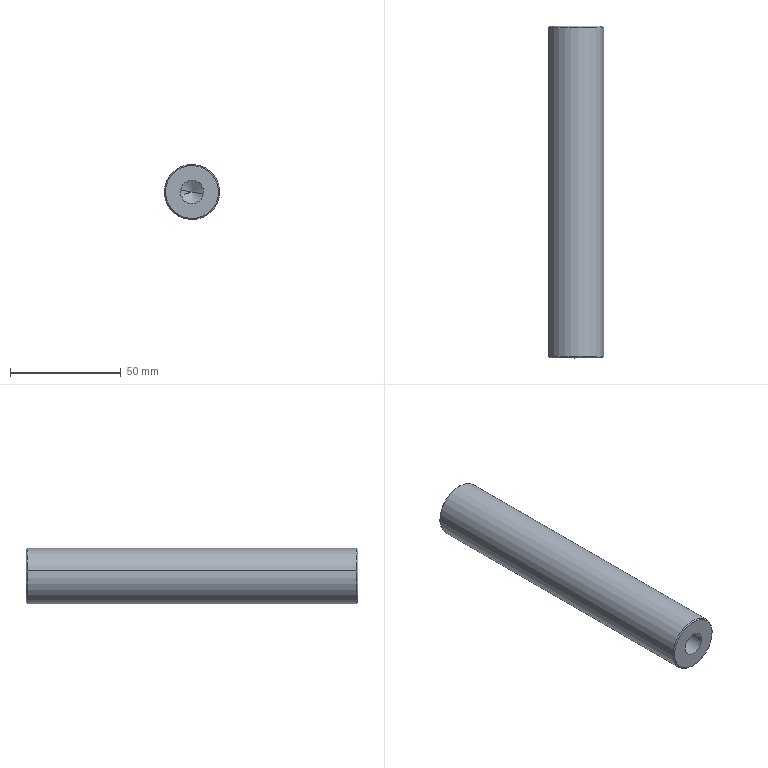Component | SolidWorks | 002AS-20130718-1_011A-20130717-4 | 1 solid | 16 faces | box 25 x 150 x 25 mm | volume 68494 mm3 | cone 8 | cylinder 6 | plane 2 | commonest cylinder face diameters 10.5 x4 25 x2
build123d program:
from build123d import *

# Parameters (mm, degrees)
SKETCH1_R                  = 12.5
BOSS_EXTRUDE1_DEPTH        = 150
M12X1_5_TAPPED_HOLE1_D     = 10.5
M12X1_5_TAPPED_HOLE1_DEPTH = 28.5
M12X1_5_TAPPED_HOLE1_TIP   = 3.155
M12X1_5_TAPPED_HOLE2_D     = 10.5
M12X1_5_TAPPED_HOLE2_DEPTH = 28.5
M12X1_5_TAPPED_HOLE2_TIP   = 3.155
CHAMFER1_SIZE              = 0.5


with BuildPart() as part:
    # Sketch1 → Boss-Extrude1 (new body)
    with BuildSketch(Plane(origin=(0, 0, 0), x_dir=(1, 0, 0), z_dir=(0, 1, 0))):
        with Locations(Location((0, 0, 0), (0, 0, 270))):
            Circle(SKETCH1_R)
    extrude(amount=BOSS_EXTRUDE1_DEPTH)

    # M12x1.5 Tapped Hole1
    with Locations(Plane.ZX.offset(150)):
        with Locations((0, 0)):
            Hole(M12X1_5_TAPPED_HOLE1_D / 2, depth=M12X1_5_TAPPED_HOLE1_DEPTH)
            with Locations((0, 0, -(M12X1_5_TAPPED_HOLE1_DEPTH + M12X1_5_TAPPED_HOLE1_TIP / 2))):  # 118° drill point
                Cone(0, M12X1_5_TAPPED_HOLE1_D / 2, M12X1_5_TAPPED_HOLE1_TIP, mode=Mode.SUBTRACT)

    # M12x1.5 Tapped Hole2
    with Locations(Plane(origin=(0, 0, 0), x_dir=(0, 0, -1), z_dir=(0, -1, 0))):
        with Locations((0, 0)):
            Hole(M12X1_5_TAPPED_HOLE2_D / 2, depth=M12X1_5_TAPPED_HOLE2_DEPTH)
            with Locations((0, 0, -(M12X1_5_TAPPED_HOLE2_DEPTH + M12X1_5_TAPPED_HOLE2_TIP / 2))):  # 118° drill point
                Cone(0, M12X1_5_TAPPED_HOLE2_D / 2, M12X1_5_TAPPED_HOLE2_TIP, mode=Mode.SUBTRACT)

    # Chamfer1
    chamfer1_edges = [part.edges().sort_by_distance(p)[0] for p in [
        (0, 0, -12.5),
        (0, 150, -12.5),
    ]]
    chamfer(chamfer1_edges, length=CHAMFER1_SIZE)


solid = part.part

# Placed as in the assembly
solid = solid.moved(Location((-292.1, 427.678, 29.291), (0, 0, 0)))
STEP:
#1=CARTESIAN_POINT('',(-11.036,16.838,1.066));
#2=VERTEX_POINT('',#1);
#3=CARTESIAN_POINT('',(-11.964,16.838,1.24));
#4=VERTEX_POINT('',#3);
#5=CARTESIAN_POINT('',(-11.5,16.838,1.153));
#6=DIRECTION('',(-0.,-1.,0.));
#7=DIRECTION('',(-0.9828,0.,0.1846));
#8=AXIS2_PLACEMENT_3D('',#5,#6,#7);
#9=CIRCLE('',#8,0.4724);
#10=EDGE_CURVE('',#2,#4,#9,.T.);
#11=ORIENTED_EDGE('',*,*,#10,.F.);
#12=CARTESIAN_POINT('',(-11.016,16.857,1.062));
#13=VERTEX_POINT('',#12);
#14=CARTESIAN_POINT('',(-11.016,16.857,1.062));
#15=DIRECTION('',(0.695,0.7071,-0.1305));
#16=VECTOR('',#15,39.37);
#17=LINE('',#14,#16);
#18=EDGE_CURVE('',#2,#13,#17,.T.);
#19=ORIENTED_EDGE('',*,*,#18,.T.);
#20=CARTESIAN_POINT('',(-11.984,16.857,1.244));
#21=VERTEX_POINT('',#20);
#22=CARTESIAN_POINT('',(-11.5,16.857,1.153));
#23=DIRECTION('',(0.,1.,-0.));
#24=DIRECTION('',(-0.9828,0.,0.1846));
#25=AXIS2_PLACEMENT_3D('',#22,#23,#24);
#26=CIRCLE('',#25,0.4921);
#27=EDGE_CURVE('',#21,#13,#26,.T.);
#28=ORIENTED_EDGE('',*,*,#27,.F.);
#29=CARTESIAN_POINT('',(-11.984,16.857,1.244));
#30=DIRECTION('',(-0.695,0.7071,0.1305));
#31=VECTOR('',#30,39.37);
#32=LINE('',#29,#31);
#33=EDGE_CURVE('',#4,#21,#32,.T.);
#34=ORIENTED_EDGE('',*,*,#33,.F.);
#35=EDGE_LOOP('',(#11,#19,#28,#34));
#36=FACE_OUTER_BOUND('',#35,.T.);
#37=CARTESIAN_POINT('',(-11.5,16.857,1.153));
#38=DIRECTION('',(0.,1.,-0.));
#39=DIRECTION('',(-0.9828,0.,0.1846));
#40=AXIS2_PLACEMENT_3D('',#37,#38,#39);
#41=CONICAL_SURFACE('',#40,0.4921,0.7854);
#42=ADVANCED_FACE('',(#36),#41,.T.);
#43=CARTESIAN_POINT('',(-11.964,22.743,1.24));
#44=VERTEX_POINT('',#43);
#45=CARTESIAN_POINT('',(-11.036,22.743,1.066));
#46=VERTEX_POINT('',#45);
#47=CARTESIAN_POINT('',(-11.5,22.743,1.153));
#48=DIRECTION('',(0.,1.,-0.));
#49=DIRECTION('',(-0.9828,0.,0.1846));
#50=AXIS2_PLACEMENT_3D('',#47,#48,#49);
#51=CIRCLE('',#50,0.4724);
#52=EDGE_CURVE('',#44,#46,#51,.T.);
#53=ORIENTED_EDGE('',*,*,#52,.F.);
#54=CARTESIAN_POINT('',(-11.984,22.724,1.244));
#55=VERTEX_POINT('',#54);
#56=CARTESIAN_POINT('',(-11.964,22.743,1.24));
#57=DIRECTION('',(-0.695,-0.7071,0.1305));
#58=VECTOR('',#57,39.37);
#59=LINE('',#56,#58);
#60=EDGE_CURVE('',#44,#55,#59,.T.);
#61=ORIENTED_EDGE('',*,*,#60,.T.);
#62=CARTESIAN_POINT('',(-11.016,22.724,1.062));
#63=VERTEX_POINT('',#62);
#64=CARTESIAN_POINT('',(-11.5,22.724,1.153));
#65=DIRECTION('',(-0.,-1.,0.));
#66=DIRECTION('',(-0.9828,0.,0.1846));
#67=AXIS2_PLACEMENT_3D('',#64,#65,#66);
#68=CIRCLE('',#67,0.4921);
#69=EDGE_CURVE('',#63,#55,#68,.T.);
#70=ORIENTED_EDGE('',*,*,#69,.F.);
#71=CARTESIAN_POINT('',(-11.036,22.743,1.066));
#72=DIRECTION('',(0.695,-0.7071,-0.1305));
#73=VECTOR('',#72,39.37);
#74=LINE('',#71,#73);
#75=EDGE_CURVE('',#46,#63,#74,.T.);
#76=ORIENTED_EDGE('',*,*,#75,.F.);
#77=EDGE_LOOP('',(#53,#61,#70,#76));
#78=FACE_OUTER_BOUND('',#77,.T.);
#79=CARTESIAN_POINT('',(-11.5,22.743,1.153));
#80=DIRECTION('',(-0.,-1.,0.));
#81=DIRECTION('',(0.9828,0.,-0.1846));
#82=AXIS2_PLACEMENT_3D('',#79,#80,#81);
#83=CONICAL_SURFACE('',#82,0.4724,0.7854);
#84=ADVANCED_FACE('',(#78),#83,.T.);
#85=CARTESIAN_POINT('',(-11.703,17.96,1.191));
#86=VERTEX_POINT('',#85);
#87=CARTESIAN_POINT('',(-11.297,17.96,1.115));
#88=VERTEX_POINT('',#87);
#89=CARTESIAN_POINT('',(-11.5,17.96,1.153));
#90=DIRECTION('',(-0.,-1.,0.));
#91=DIRECTION('',(0.9828,0.,-0.1846));
#92=AXIS2_PLACEMENT_3D('',#89,#90,#91);
#93=CIRCLE('',#92,0.2067);
#94=EDGE_CURVE('',#86,#88,#93,.T.);
#95=ORIENTED_EDGE('',*,*,#94,.F.);
#96=CARTESIAN_POINT('',(-11.703,16.838,1.191));
#97=VERTEX_POINT('',#96);
#98=CARTESIAN_POINT('',(-11.703,16.838,1.191));
#99=DIRECTION('',(-0.,-1.,0.));
#100=VECTOR('',#99,39.37);
#101=LINE('',#98,#100);
#102=EDGE_CURVE('',#86,#97,#101,.T.);
#103=ORIENTED_EDGE('',*,*,#102,.T.);
#104=CARTESIAN_POINT('',(-11.297,16.838,1.115));
#105=VERTEX_POINT('',#104);
#106=CARTESIAN_POINT('',(-11.5,16.838,1.153));
#107=DIRECTION('',(-0.,-1.,0.));
#108=DIRECTION('',(0.9828,0.,-0.1846));
#109=AXIS2_PLACEMENT_3D('',#106,#107,#108);
#110=CIRCLE('',#109,0.2067);
#111=EDGE_CURVE('',#97,#105,#110,.T.);
#112=ORIENTED_EDGE('',*,*,#111,.T.);
#113=CARTESIAN_POINT('',(-11.297,16.838,1.115));
#114=DIRECTION('',(-0.,-1.,0.));
#115=VECTOR('',#114,39.37);
#116=LINE('',#113,#115);
#117=EDGE_CURVE('',#88,#105,#116,.T.);
#118=ORIENTED_EDGE('',*,*,#117,.F.);
#119=EDGE_LOOP('',(#95,#103,#112,#118));
#120=FACE_OUTER_BOUND('',#119,.T.);
#121=CARTESIAN_POINT('',(-11.5,16.838,1.153));
#122=DIRECTION('',(-0.,-1.,0.));
#123=DIRECTION('',(0.9828,0.,-0.1846));
#124=AXIS2_PLACEMENT_3D('',#121,#122,#123);
#125=CYLINDRICAL_SURFACE('',#124,0.2067);
#126=ADVANCED_FACE('',(#120),#125,.F.);
#127=CARTESIAN_POINT('',(-11.5,18.084,1.153));
#128=VERTEX_POINT('',#127);
#129=CARTESIAN_POINT('',(-11.297,17.96,1.115));
#130=DIRECTION('',(0.8424,-0.515,-0.1582));
#131=VECTOR('',#130,39.37);
#132=LINE('',#129,#131);
#133=EDGE_CURVE('',#128,#88,#132,.T.);
#134=ORIENTED_EDGE('',*,*,#133,.F.);
#135=CARTESIAN_POINT('',(-11.703,17.96,1.191));
#136=DIRECTION('',(-0.8424,-0.515,0.1582));
#137=VECTOR('',#136,39.37);
#138=LINE('',#135,#137);
#139=EDGE_CURVE('',#128,#86,#138,.T.);
#140=ORIENTED_EDGE('',*,*,#139,.T.);
#141=ORIENTED_EDGE('',*,*,#94,.T.);
#142=EDGE_LOOP('',(#134,#140,#141));
#143=FACE_OUTER_BOUND('',#142,.T.);
#144=CARTESIAN_POINT('',(-11.5,17.96,1.153));
#145=DIRECTION('',(-0.,-1.,0.));
#146=DIRECTION('',(0.9828,0.,-0.1846));
#147=AXIS2_PLACEMENT_3D('',#144,#145,#146);
#148=CONICAL_SURFACE('',#147,0.2067,1.03);
#149=ADVANCED_FACE('',(#143),#148,.F.);
#150=CARTESIAN_POINT('',(-11.297,21.621,1.115));
#151=VERTEX_POINT('',#150);
#152=CARTESIAN_POINT('',(-11.703,21.621,1.191));
#153=VERTEX_POINT('',#152);
#154=CARTESIAN_POINT('',(-11.5,21.621,1.153));
#155=DIRECTION('',(0.,1.,-0.));
#156=DIRECTION('',(-0.9828,0.,0.1846));
#157=AXIS2_PLACEMENT_3D('',#154,#155,#156);
#158=CIRCLE('',#157,0.2067);
#159=EDGE_CURVE('',#151,#153,#158,.T.);
#160=ORIENTED_EDGE('',*,*,#159,.F.);
#161=CARTESIAN_POINT('',(-11.297,22.743,1.115));
#162=VERTEX_POINT('',#161);
#163=CARTESIAN_POINT('',(-11.297,22.743,1.115));
#164=DIRECTION('',(0.,1.,-0.));
#165=VECTOR('',#164,39.37);
#166=LINE('',#163,#165);
#167=EDGE_CURVE('',#151,#162,#166,.T.);
#168=ORIENTED_EDGE('',*,*,#167,.T.);
#169=CARTESIAN_POINT('',(-11.703,22.743,1.191));
#170=VERTEX_POINT('',#169);
#171=CARTESIAN_POINT('',(-11.5,22.743,1.153));
#172=DIRECTION('',(0.,1.,-0.));
#173=DIRECTION('',(-0.9828,0.,0.1846));
#174=AXIS2_PLACEMENT_3D('',#171,#172,#173);
#175=CIRCLE('',#174,0.2067);
#176=EDGE_CURVE('',#162,#170,#175,.T.);
#177=ORIENTED_EDGE('',*,*,#176,.T.);
#178=CARTESIAN_POINT('',(-11.703,22.743,1.191));
#179=DIRECTION('',(0.,1.,-0.));
#180=VECTOR('',#179,39.37);
#181=LINE('',#178,#180);
#182=EDGE_CURVE('',#153,#170,#181,.T.);
#183=ORIENTED_EDGE('',*,*,#182,.F.);
#184=EDGE_LOOP('',(#160,#168,#177,#183));
#185=FACE_OUTER_BOUND('',#184,.T.);
#186=CARTESIAN_POINT('',(-11.5,22.743,1.153));
#187=DIRECTION('',(0.,1.,-0.));
#188=DIRECTION('',(-0.9828,0.,0.1846));
#189=AXIS2_PLACEMENT_3D('',#186,#187,#188);
#190=CYLINDRICAL_SURFACE('',#189,0.2067);
#191=ADVANCED_FACE('',(#185),#190,.F.);
#192=CARTESIAN_POINT('',(-11.5,21.497,1.153));
#193=VERTEX_POINT('',#192);
#194=CARTESIAN_POINT('',(-11.703,21.621,1.191));
#195=DIRECTION('',(-0.8424,0.515,0.1582));
#196=VECTOR('',#195,39.37);
#197=LINE('',#194,#196);
#198=EDGE_CURVE('',#193,#153,#197,.T.);
#199=ORIENTED_EDGE('',*,*,#198,.F.);
#200=CARTESIAN_POINT('',(-11.297,21.621,1.115));
#201=DIRECTION('',(0.8424,0.515,-0.1582));
#202=VECTOR('',#201,39.37);
#203=LINE('',#200,#202);
#204=EDGE_CURVE('',#193,#151,#203,.T.);
#205=ORIENTED_EDGE('',*,*,#204,.T.);
#206=ORIENTED_EDGE('',*,*,#159,.T.);
#207=EDGE_LOOP('',(#199,#205,#206));
#208=FACE_OUTER_BOUND('',#207,.T.);
#209=CARTESIAN_POINT('',(-11.5,21.621,1.153));
#210=DIRECTION('',(0.,1.,-0.));
#211=DIRECTION('',(-0.9828,0.,0.1846));
#212=AXIS2_PLACEMENT_3D('',#209,#210,#211);
#213=CONICAL_SURFACE('',#212,0.2067,1.03);
#214=ADVANCED_FACE('',(#208),#213,.F.);
#215=ORIENTED_EDGE('',*,*,#69,.T.);
#216=CARTESIAN_POINT('',(-11.984,22.743,1.244));
#217=DIRECTION('',(-0.,-1.,0.));
#218=VECTOR('',#217,39.37);
#219=LINE('',#216,#218);
#220=EDGE_CURVE('',#55,#21,#219,.T.);
#221=ORIENTED_EDGE('',*,*,#220,.T.);
#222=ORIENTED_EDGE('',*,*,#27,.T.);
#223=CARTESIAN_POINT('',(-11.016,22.743,1.062));
#224=DIRECTION('',(-0.,-1.,0.));
#225=VECTOR('',#224,39.37);
#226=LINE('',#223,#225);
#227=EDGE_CURVE('',#63,#13,#226,.T.);
#228=ORIENTED_EDGE('',*,*,#227,.F.);
#229=EDGE_LOOP('',(#215,#221,#222,#228));
#230=FACE_OUTER_BOUND('',#229,.T.);
#231=CARTESIAN_POINT('',(-11.5,22.743,1.153));
#232=DIRECTION('',(-0.,-1.,0.));
#233=DIRECTION('',(0.9828,0.,-0.1846));
#234=AXIS2_PLACEMENT_3D('',#231,#232,#233);
#235=CYLINDRICAL_SURFACE('',#234,0.4921);
#236=ADVANCED_FACE('',(#230),#235,.T.);
#237=ORIENTED_EDGE('',*,*,#220,.F.);
#238=CARTESIAN_POINT('',(-11.5,22.724,1.153));
#239=DIRECTION('',(-0.,-1.,0.));
#240=DIRECTION('',(-0.9828,0.,0.1846));
#241=AXIS2_PLACEMENT_3D('',#238,#239,#240);
#242=CIRCLE('',#241,0.4921);
#243=EDGE_CURVE('',#55,#63,#242,.T.);
#244=ORIENTED_EDGE('',*,*,#243,.T.);
#245=ORIENTED_EDGE('',*,*,#227,.T.);
#246=CARTESIAN_POINT('',(-11.5,16.857,1.153));
#247=DIRECTION('',(0.,1.,-0.));
#248=DIRECTION('',(-0.9828,0.,0.1846));
#249=AXIS2_PLACEMENT_3D('',#246,#247,#248);
#250=CIRCLE('',#249,0.4921);
#251=EDGE_CURVE('',#13,#21,#250,.T.);
#252=ORIENTED_EDGE('',*,*,#251,.T.);
#253=EDGE_LOOP('',(#237,#244,#245,#252));
#254=FACE_OUTER_BOUND('',#253,.T.);
#255=CARTESIAN_POINT('',(-11.5,22.743,1.153));
#256=DIRECTION('',(-0.,-1.,0.));
#257=DIRECTION('',(0.9828,0.,-0.1846));
#258=AXIS2_PLACEMENT_3D('',#255,#256,#257);
#259=CYLINDRICAL_SURFACE('',#258,0.4921);
#260=ADVANCED_FACE('',(#254),#259,.T.);
#261=CARTESIAN_POINT('',(-11.5,22.743,1.153));
#262=DIRECTION('',(0.,1.,-0.));
#263=DIRECTION('',(-0.9828,0.,0.1846));
#264=AXIS2_PLACEMENT_3D('',#261,#262,#263);
#265=CIRCLE('',#264,0.4724);
#266=EDGE_CURVE('',#46,#44,#265,.T.);
#267=ORIENTED_EDGE('',*,*,#266,.T.);
#268=ORIENTED_EDGE('',*,*,#52,.T.);
#269=EDGE_LOOP('',(#267,#268));
#270=FACE_OUTER_BOUND('',#269,.T.);
#271=CARTESIAN_POINT('',(-11.5,22.743,1.153));
#272=DIRECTION('',(0.,1.,-0.));
#273=DIRECTION('',(-0.9828,0.,0.1846));
#274=AXIS2_PLACEMENT_3D('',#271,#272,#273);
#275=CIRCLE('',#274,0.2067);
#276=EDGE_CURVE('',#170,#162,#275,.T.);
#277=ORIENTED_EDGE('',*,*,#276,.F.);
#278=ORIENTED_EDGE('',*,*,#176,.F.);
#279=EDGE_LOOP('',(#277,#278));
#280=FACE_BOUND('',#279,.T.);
#281=CARTESIAN_POINT('',(-11.5,22.743,1.153));
#282=DIRECTION('',(0.,1.,-0.));
#283=DIRECTION('',(-0.9828,0.,0.1846));
#284=AXIS2_PLACEMENT_3D('',#281,#282,#283);
#285=PLANE('',#284);
#286=ADVANCED_FACE('',(#270,#280),#285,.T.);
#287=CARTESIAN_POINT('',(-11.5,16.838,1.153));
#288=DIRECTION('',(-0.,-1.,0.));
#289=DIRECTION('',(-0.9828,0.,0.1846));
#290=AXIS2_PLACEMENT_3D('',#287,#288,#289);
#291=CIRCLE('',#290,0.4724);
#292=EDGE_CURVE('',#4,#2,#291,.T.);
#293=ORIENTED_EDGE('',*,*,#292,.T.);
#294=ORIENTED_EDGE('',*,*,#10,.T.);
#295=EDGE_LOOP('',(#293,#294));
#296=FACE_OUTER_BOUND('',#295,.T.);
#297=CARTESIAN_POINT('',(-11.5,16.838,1.153));
#298=DIRECTION('',(-0.,-1.,0.));
#299=DIRECTION('',(0.9828,0.,-0.1846));
#300=AXIS2_PLACEMENT_3D('',#297,#298,#299);
#301=CIRCLE('',#300,0.2067);
#302=EDGE_CURVE('',#105,#97,#301,.T.);
#303=ORIENTED_EDGE('',*,*,#302,.F.);
#304=ORIENTED_EDGE('',*,*,#111,.F.);
#305=EDGE_LOOP('',(#303,#304));
#306=FACE_BOUND('',#305,.T.);
#307=CARTESIAN_POINT('',(-11.5,16.838,1.153));
#308=DIRECTION('',(0.,1.,-0.));
#309=DIRECTION('',(-0.9828,0.,0.1846));
#310=AXIS2_PLACEMENT_3D('',#307,#308,#309);
#311=PLANE('',#310);
#312=ADVANCED_FACE('',(#296,#306),#311,.F.);
#313=ORIENTED_EDGE('',*,*,#204,.F.);
#314=ORIENTED_EDGE('',*,*,#198,.T.);
#315=CARTESIAN_POINT('',(-11.5,21.621,1.153));
#316=DIRECTION('',(0.,1.,-0.));
#317=DIRECTION('',(-0.9828,0.,0.1846));
#318=AXIS2_PLACEMENT_3D('',#315,#316,#317);
#319=CIRCLE('',#318,0.2067);
#320=EDGE_CURVE('',#153,#151,#319,.T.);
#321=ORIENTED_EDGE('',*,*,#320,.T.);
#322=EDGE_LOOP('',(#313,#314,#321));
#323=FACE_OUTER_BOUND('',#322,.T.);
#324=CARTESIAN_POINT('',(-11.5,21.621,1.153));
#325=DIRECTION('',(0.,1.,-0.));
#326=DIRECTION('',(-0.9828,0.,0.1846));
#327=AXIS2_PLACEMENT_3D('',#324,#325,#326);
#328=CONICAL_SURFACE('',#327,0.2067,1.03);
#329=ADVANCED_FACE('',(#323),#328,.F.);
#330=ORIENTED_EDGE('',*,*,#167,.F.);
#331=ORIENTED_EDGE('',*,*,#320,.F.);
#332=ORIENTED_EDGE('',*,*,#182,.T.);
#333=ORIENTED_EDGE('',*,*,#276,.T.);
#334=EDGE_LOOP('',(#330,#331,#332,#333));
#335=FACE_OUTER_BOUND('',#334,.T.);
#336=CARTESIAN_POINT('',(-11.5,22.743,1.153));
#337=DIRECTION('',(0.,1.,-0.));
#338=DIRECTION('',(-0.9828,0.,0.1846));
#339=AXIS2_PLACEMENT_3D('',#336,#337,#338);
#340=CYLINDRICAL_SURFACE('',#339,0.2067);
#341=ADVANCED_FACE('',(#335),#340,.F.);
#342=ORIENTED_EDGE('',*,*,#139,.F.);
#343=ORIENTED_EDGE('',*,*,#133,.T.);
#344=CARTESIAN_POINT('',(-11.5,17.96,1.153));
#345=DIRECTION('',(-0.,-1.,0.));
#346=DIRECTION('',(0.9828,0.,-0.1846));
#347=AXIS2_PLACEMENT_3D('',#344,#345,#346);
#348=CIRCLE('',#347,0.2067);
#349=EDGE_CURVE('',#88,#86,#348,.T.);
#350=ORIENTED_EDGE('',*,*,#349,.T.);
#351=EDGE_LOOP('',(#342,#343,#350));
#352=FACE_OUTER_BOUND('',#351,.T.);
#353=CARTESIAN_POINT('',(-11.5,17.96,1.153));
#354=DIRECTION('',(-0.,-1.,0.));
#355=DIRECTION('',(0.9828,0.,-0.1846));
#356=AXIS2_PLACEMENT_3D('',#353,#354,#355);
#357=CONICAL_SURFACE('',#356,0.2067,1.03);
#358=ADVANCED_FACE('',(#352),#357,.F.);
#359=ORIENTED_EDGE('',*,*,#102,.F.);
#360=ORIENTED_EDGE('',*,*,#349,.F.);
#361=ORIENTED_EDGE('',*,*,#117,.T.);
#362=ORIENTED_EDGE('',*,*,#302,.T.);
#363=EDGE_LOOP('',(#359,#360,#361,#362));
#364=FACE_OUTER_BOUND('',#363,.T.);
#365=CARTESIAN_POINT('',(-11.5,16.838,1.153));
#366=DIRECTION('',(-0.,-1.,0.));
#367=DIRECTION('',(0.9828,0.,-0.1846));
#368=AXIS2_PLACEMENT_3D('',#365,#366,#367);
#369=CYLINDRICAL_SURFACE('',#368,0.2067);
#370=ADVANCED_FACE('',(#364),#369,.F.);
#371=ORIENTED_EDGE('',*,*,#60,.F.);
#372=ORIENTED_EDGE('',*,*,#266,.F.);
#373=ORIENTED_EDGE('',*,*,#75,.T.);
#374=ORIENTED_EDGE('',*,*,#243,.F.);
#375=EDGE_LOOP('',(#371,#372,#373,#374));
#376=FACE_OUTER_BOUND('',#375,.T.);
#377=CARTESIAN_POINT('',(-11.5,22.743,1.153));
#378=DIRECTION('',(-0.,-1.,0.));
#379=DIRECTION('',(0.9828,0.,-0.1846));
#380=AXIS2_PLACEMENT_3D('',#377,#378,#379);
#381=CONICAL_SURFACE('',#380,0.4724,0.7854);
#382=ADVANCED_FACE('',(#376),#381,.T.);
#383=ORIENTED_EDGE('',*,*,#18,.F.);
#384=ORIENTED_EDGE('',*,*,#292,.F.);
#385=ORIENTED_EDGE('',*,*,#33,.T.);
#386=ORIENTED_EDGE('',*,*,#251,.F.);
#387=EDGE_LOOP('',(#383,#384,#385,#386));
#388=FACE_OUTER_BOUND('',#387,.T.);
#389=CARTESIAN_POINT('',(-11.5,16.857,1.153));
#390=DIRECTION('',(0.,1.,-0.));
#391=DIRECTION('',(-0.9828,0.,0.1846));
#392=AXIS2_PLACEMENT_3D('',#389,#390,#391);
#393=CONICAL_SURFACE('',#392,0.4921,0.7854);
#394=ADVANCED_FACE('',(#388),#393,.T.);
#395=CLOSED_SHELL('',(#42,#84,#126,#149,#191,#214,#236,#260,#286,#312,#329,#341,#358,#370,#382,#394));
#396=MANIFOLD_SOLID_BREP('',#395);
#397=CARTESIAN_POINT('',(0.,0.,0.));
#398=DIRECTION('',(0.,0.,1.));
#399=DIRECTION('',(1.,0.,0.));
#400=AXIS2_PLACEMENT_3D('',#397,#398,#399);
#401=(LENGTH_UNIT()NAMED_UNIT(*)SI_UNIT($,.METRE.));
#402=LENGTH_MEASURE_WITH_UNIT(LENGTH_MEASURE(0.0254),#401);
#403=DIMENSIONAL_EXPONENTS(1.,0.,0.,0.,0.,0.,0.);
#404=(CONVERSION_BASED_UNIT('',#402)LENGTH_UNIT()NAMED_UNIT(#403));
#405=UNCERTAINTY_MEASURE_WITH_UNIT(LENGTH_MEASURE(0.00001),#404,'','');
#406=(NAMED_UNIT(*)PLANE_ANGLE_UNIT()SI_UNIT($,.RADIAN.));
#407=(NAMED_UNIT(*)SI_UNIT($,.STERADIAN.)SOLID_ANGLE_UNIT());
#408=(GEOMETRIC_REPRESENTATION_CONTEXT(3)GLOBAL_UNCERTAINTY_ASSIGNED_CONTEXT((#405))GLOBAL_UNIT_ASSIGNED_CONTEXT((#404,#406,#407))REPRESENTATION_CONTEXT('',''));
#409=ADVANCED_BREP_SHAPE_REPRESENTATION('',(#396,#400),#408);
#410=COLOUR_RGB('',0.7922,0.8196,0.9333);
#411=FILL_AREA_STYLE_COLOUR('',#410);
#412=FILL_AREA_STYLE('',(#411));
#413=SURFACE_STYLE_FILL_AREA(#412);
#414=SURFACE_SIDE_STYLE('',(#413));
#415=SURFACE_STYLE_USAGE(.BOTH.,#414);
#416=PRESENTATION_STYLE_ASSIGNMENT((#415));
#417=STYLED_ITEM('',(#416),#396);
#418=PRESENTATION_LAYER_ASSIGNMENT('','',(#417));
#419=(LENGTH_UNIT()NAMED_UNIT(*)SI_UNIT($,.METRE.));
#420=LENGTH_MEASURE_WITH_UNIT(LENGTH_MEASURE(0.0254),#419);
#421=DIMENSIONAL_EXPONENTS(1.,0.,0.,0.,0.,0.,0.);
#422=(CONVERSION_BASED_UNIT('',#420)LENGTH_UNIT()NAMED_UNIT(#421));
#423=UNCERTAINTY_MEASURE_WITH_UNIT(LENGTH_MEASURE(0.00001),#422,'','');
#424=(NAMED_UNIT(*)PLANE_ANGLE_UNIT()SI_UNIT($,.RADIAN.));
#425=(NAMED_UNIT(*)SI_UNIT($,.STERADIAN.)SOLID_ANGLE_UNIT());
#426=(GEOMETRIC_REPRESENTATION_CONTEXT(3)GLOBAL_UNCERTAINTY_ASSIGNED_CONTEXT((#423))GLOBAL_UNIT_ASSIGNED_CONTEXT((#422,#424,#425))REPRESENTATION_CONTEXT('',''));
#427=MECHANICAL_DESIGN_GEOMETRIC_PRESENTATION_REPRESENTATION('',(#417),#426);